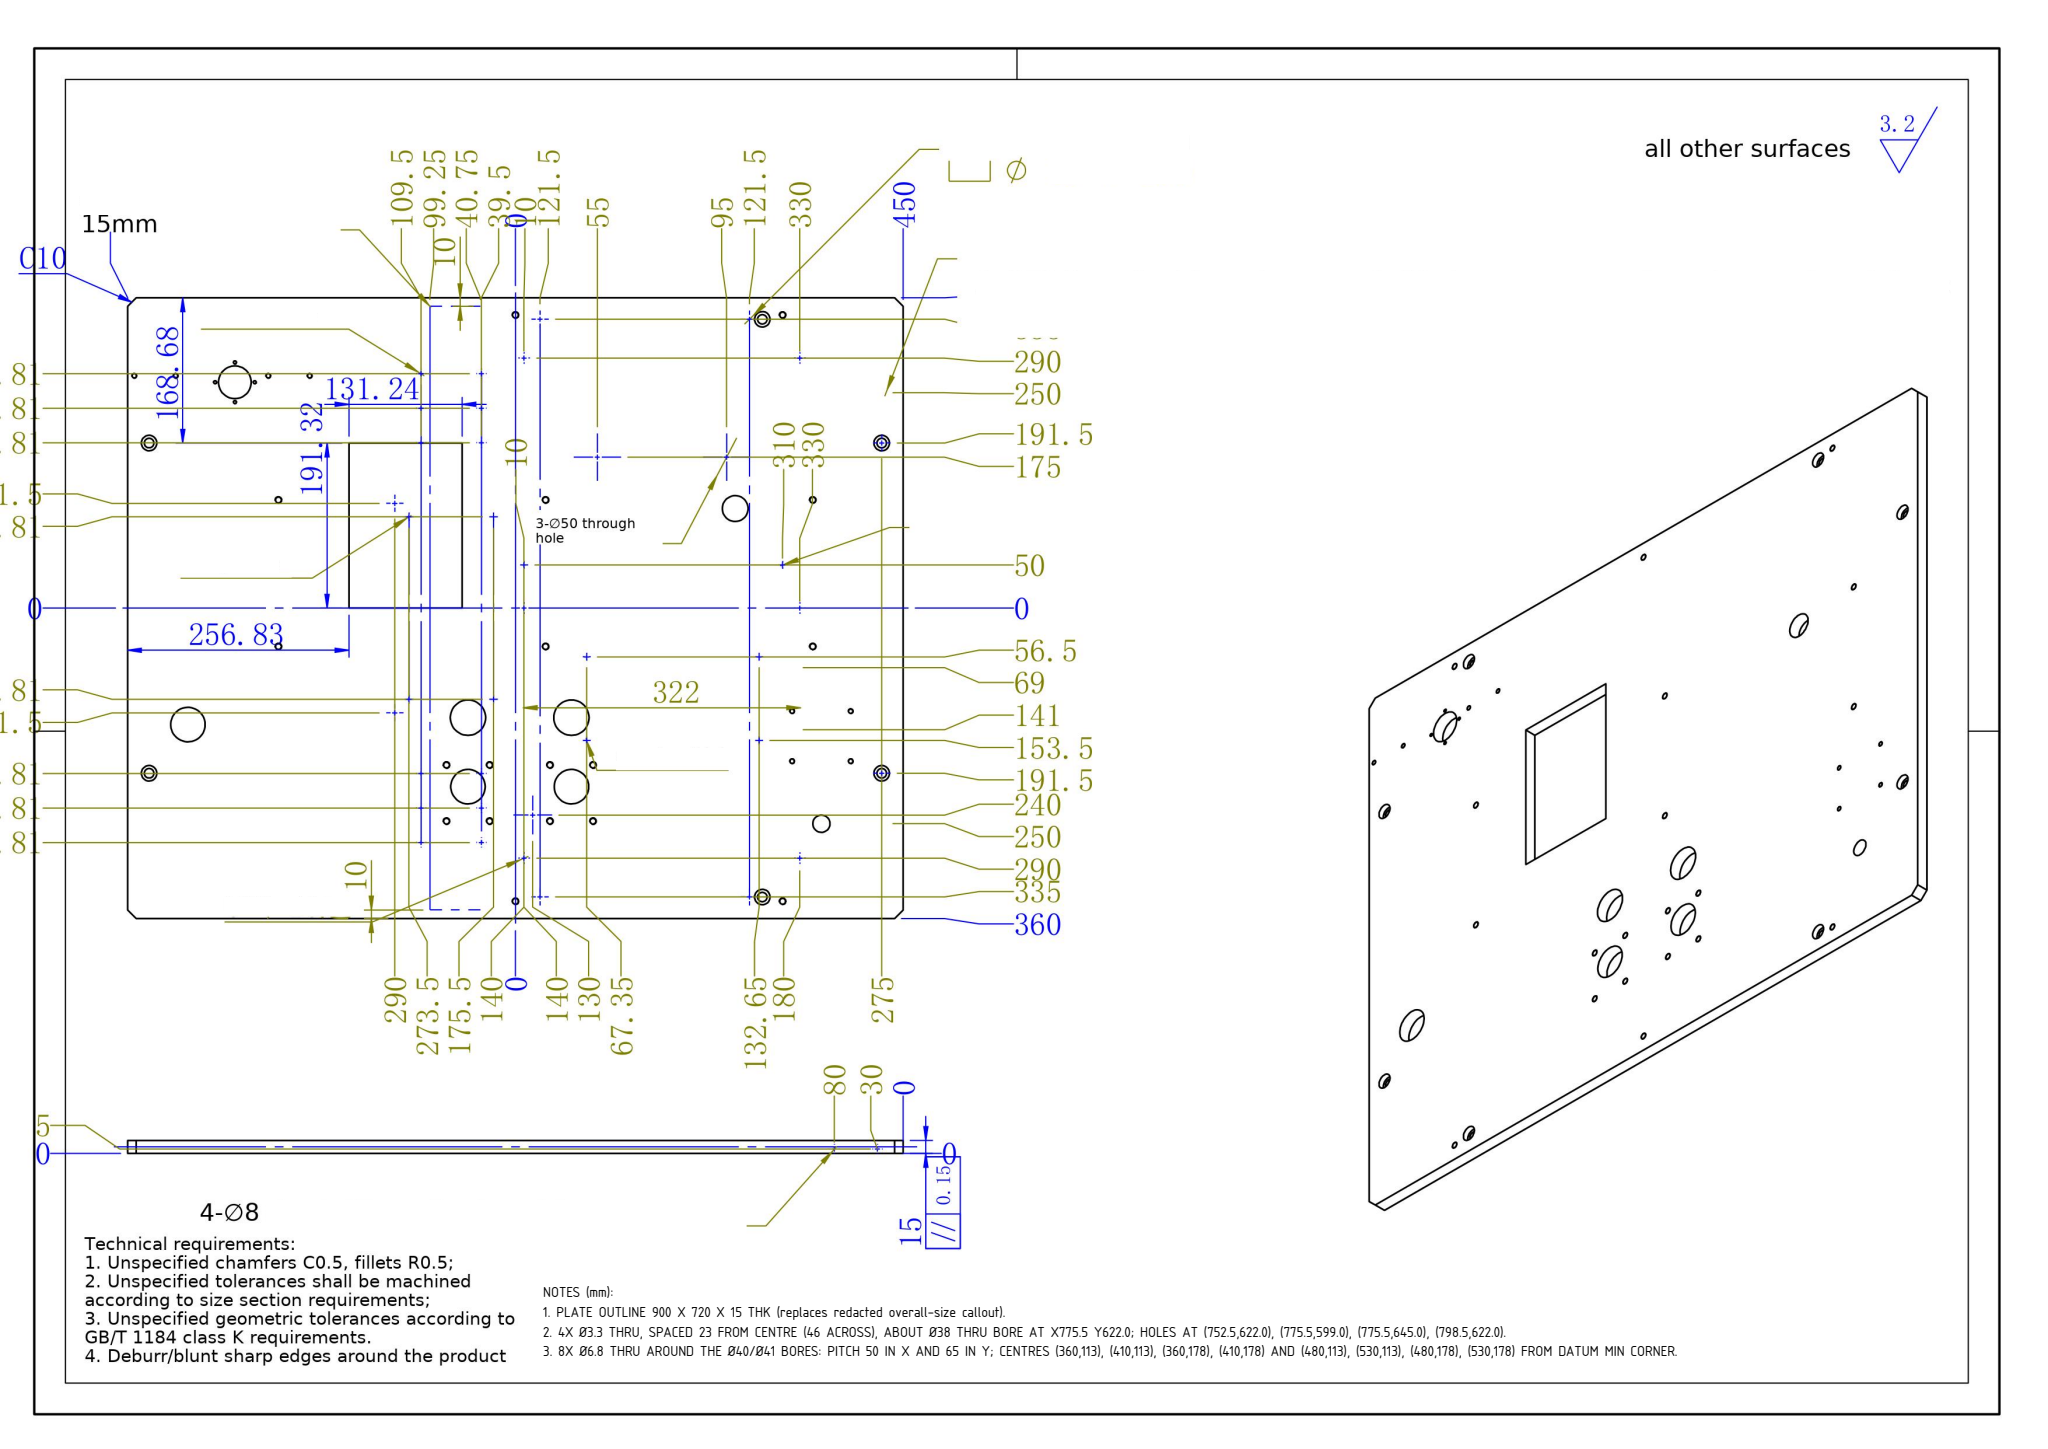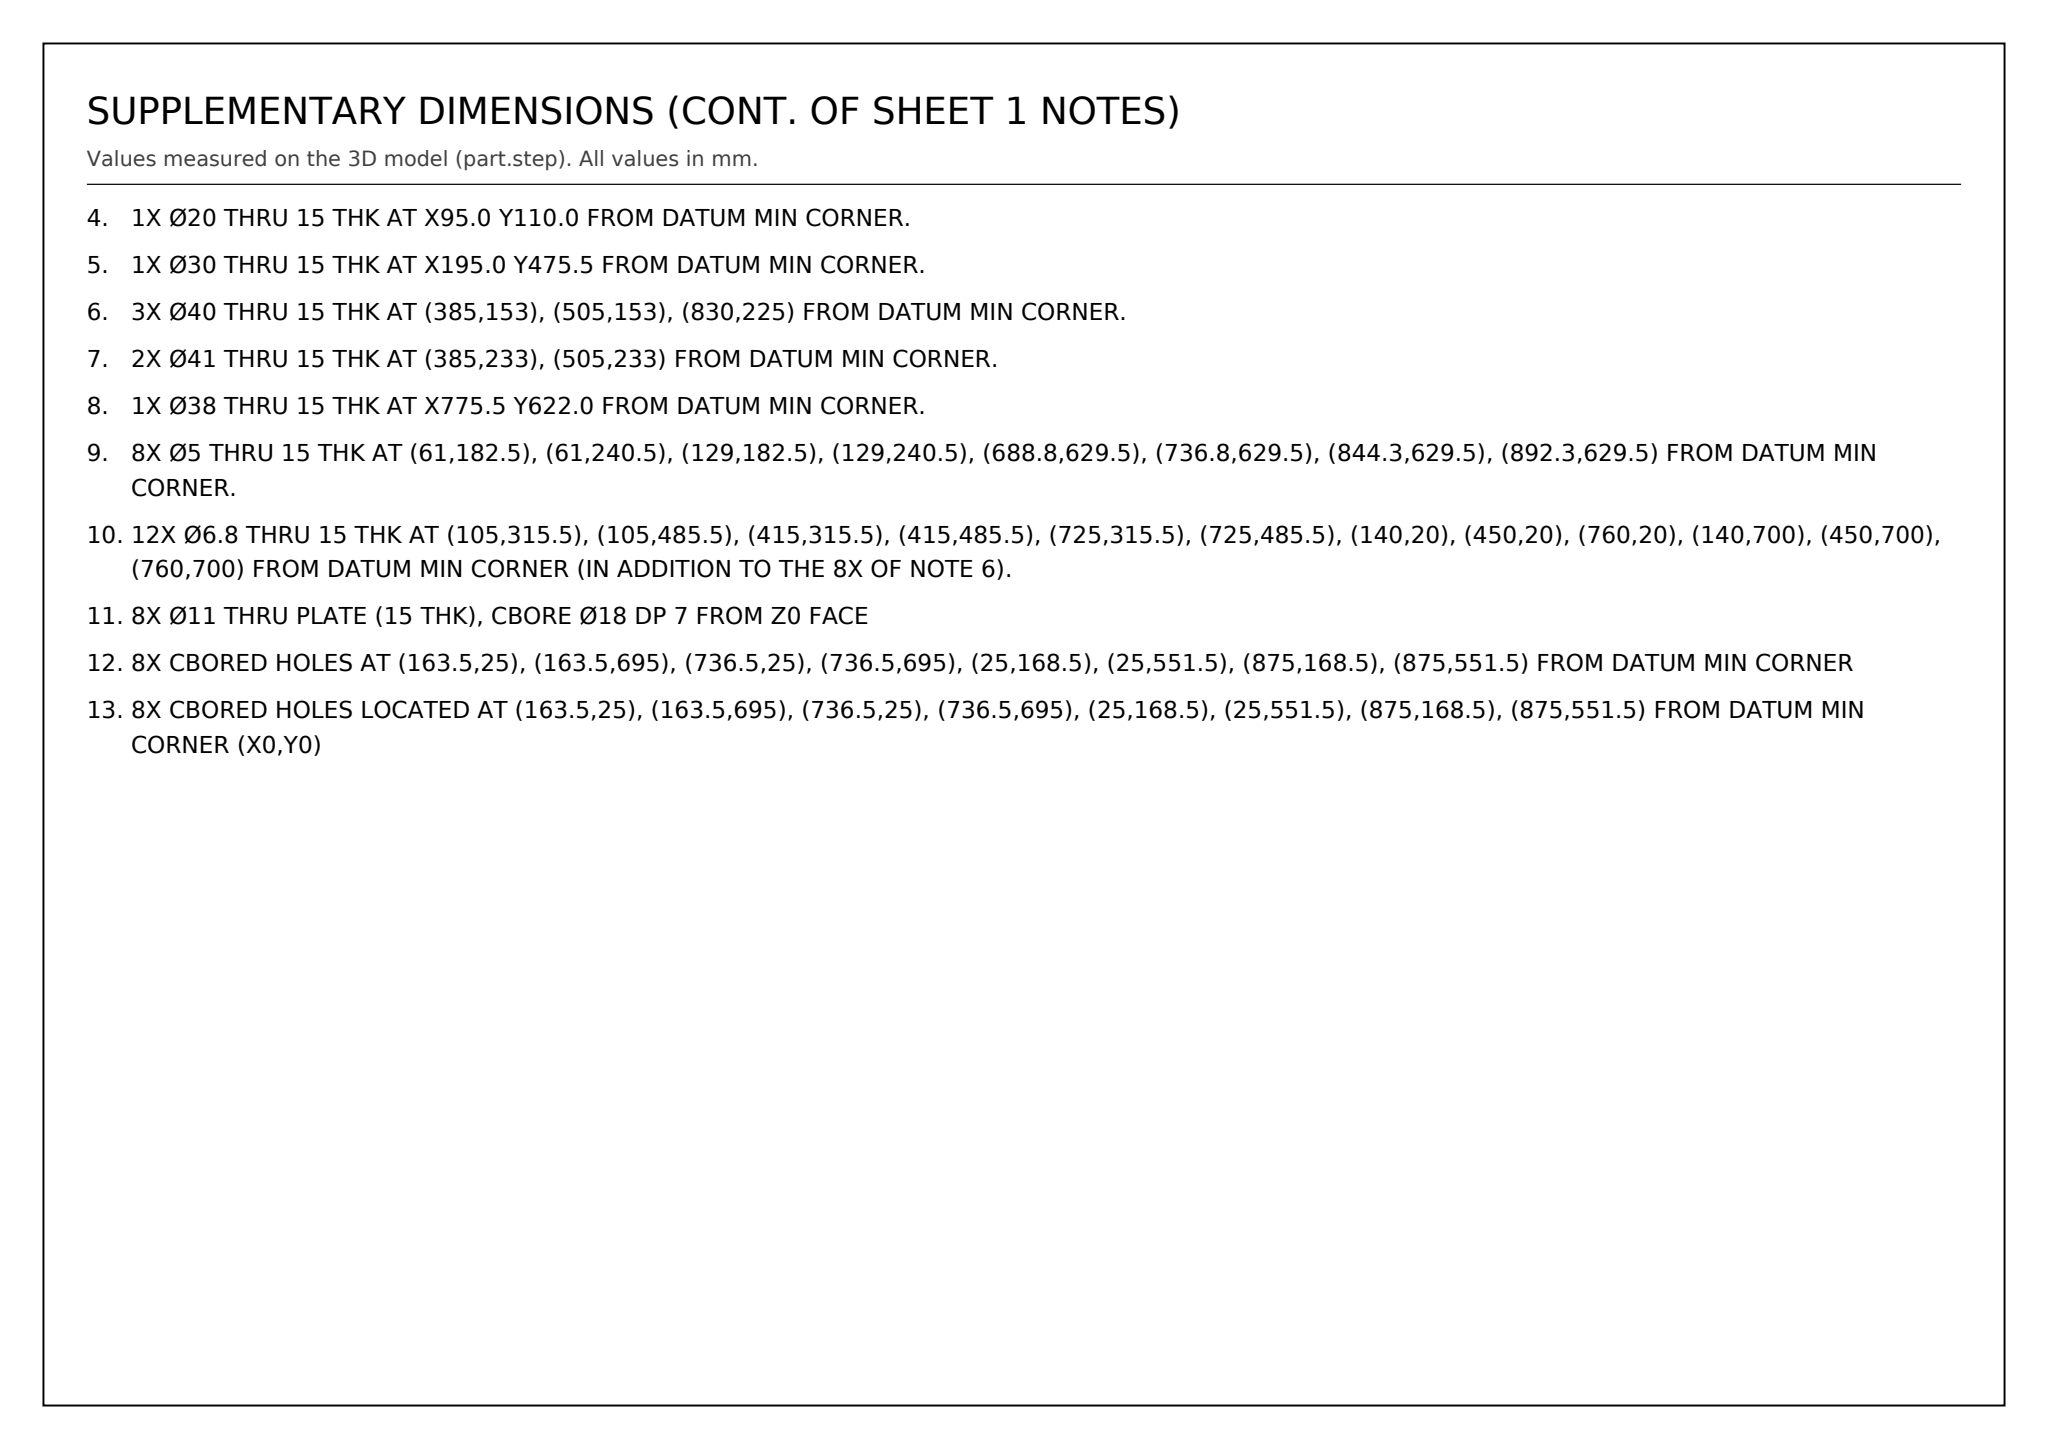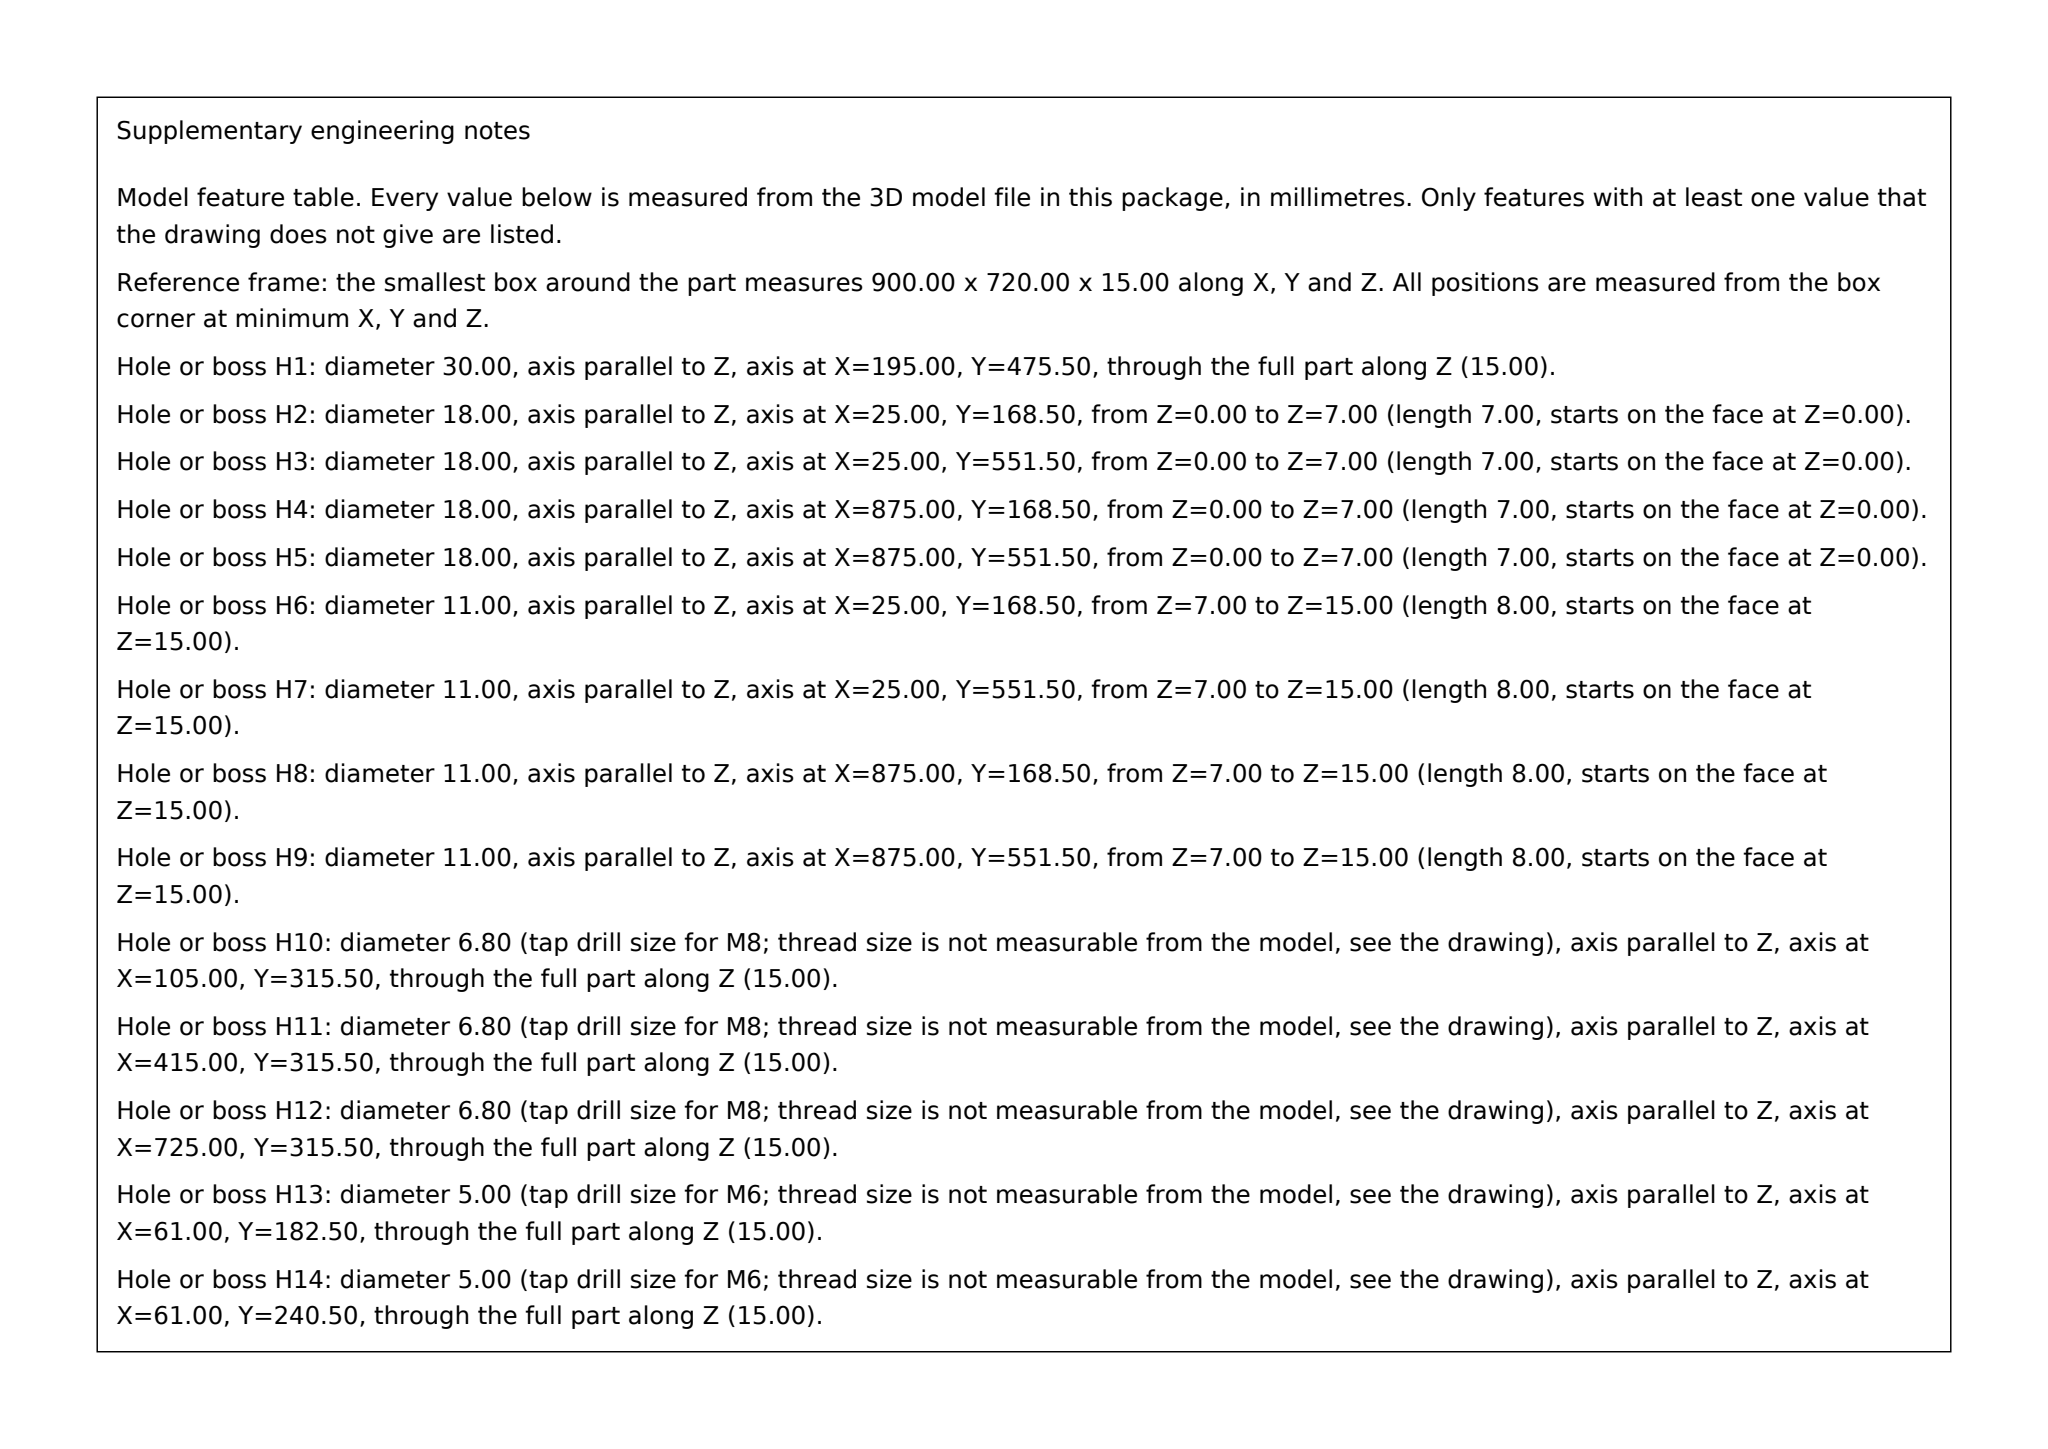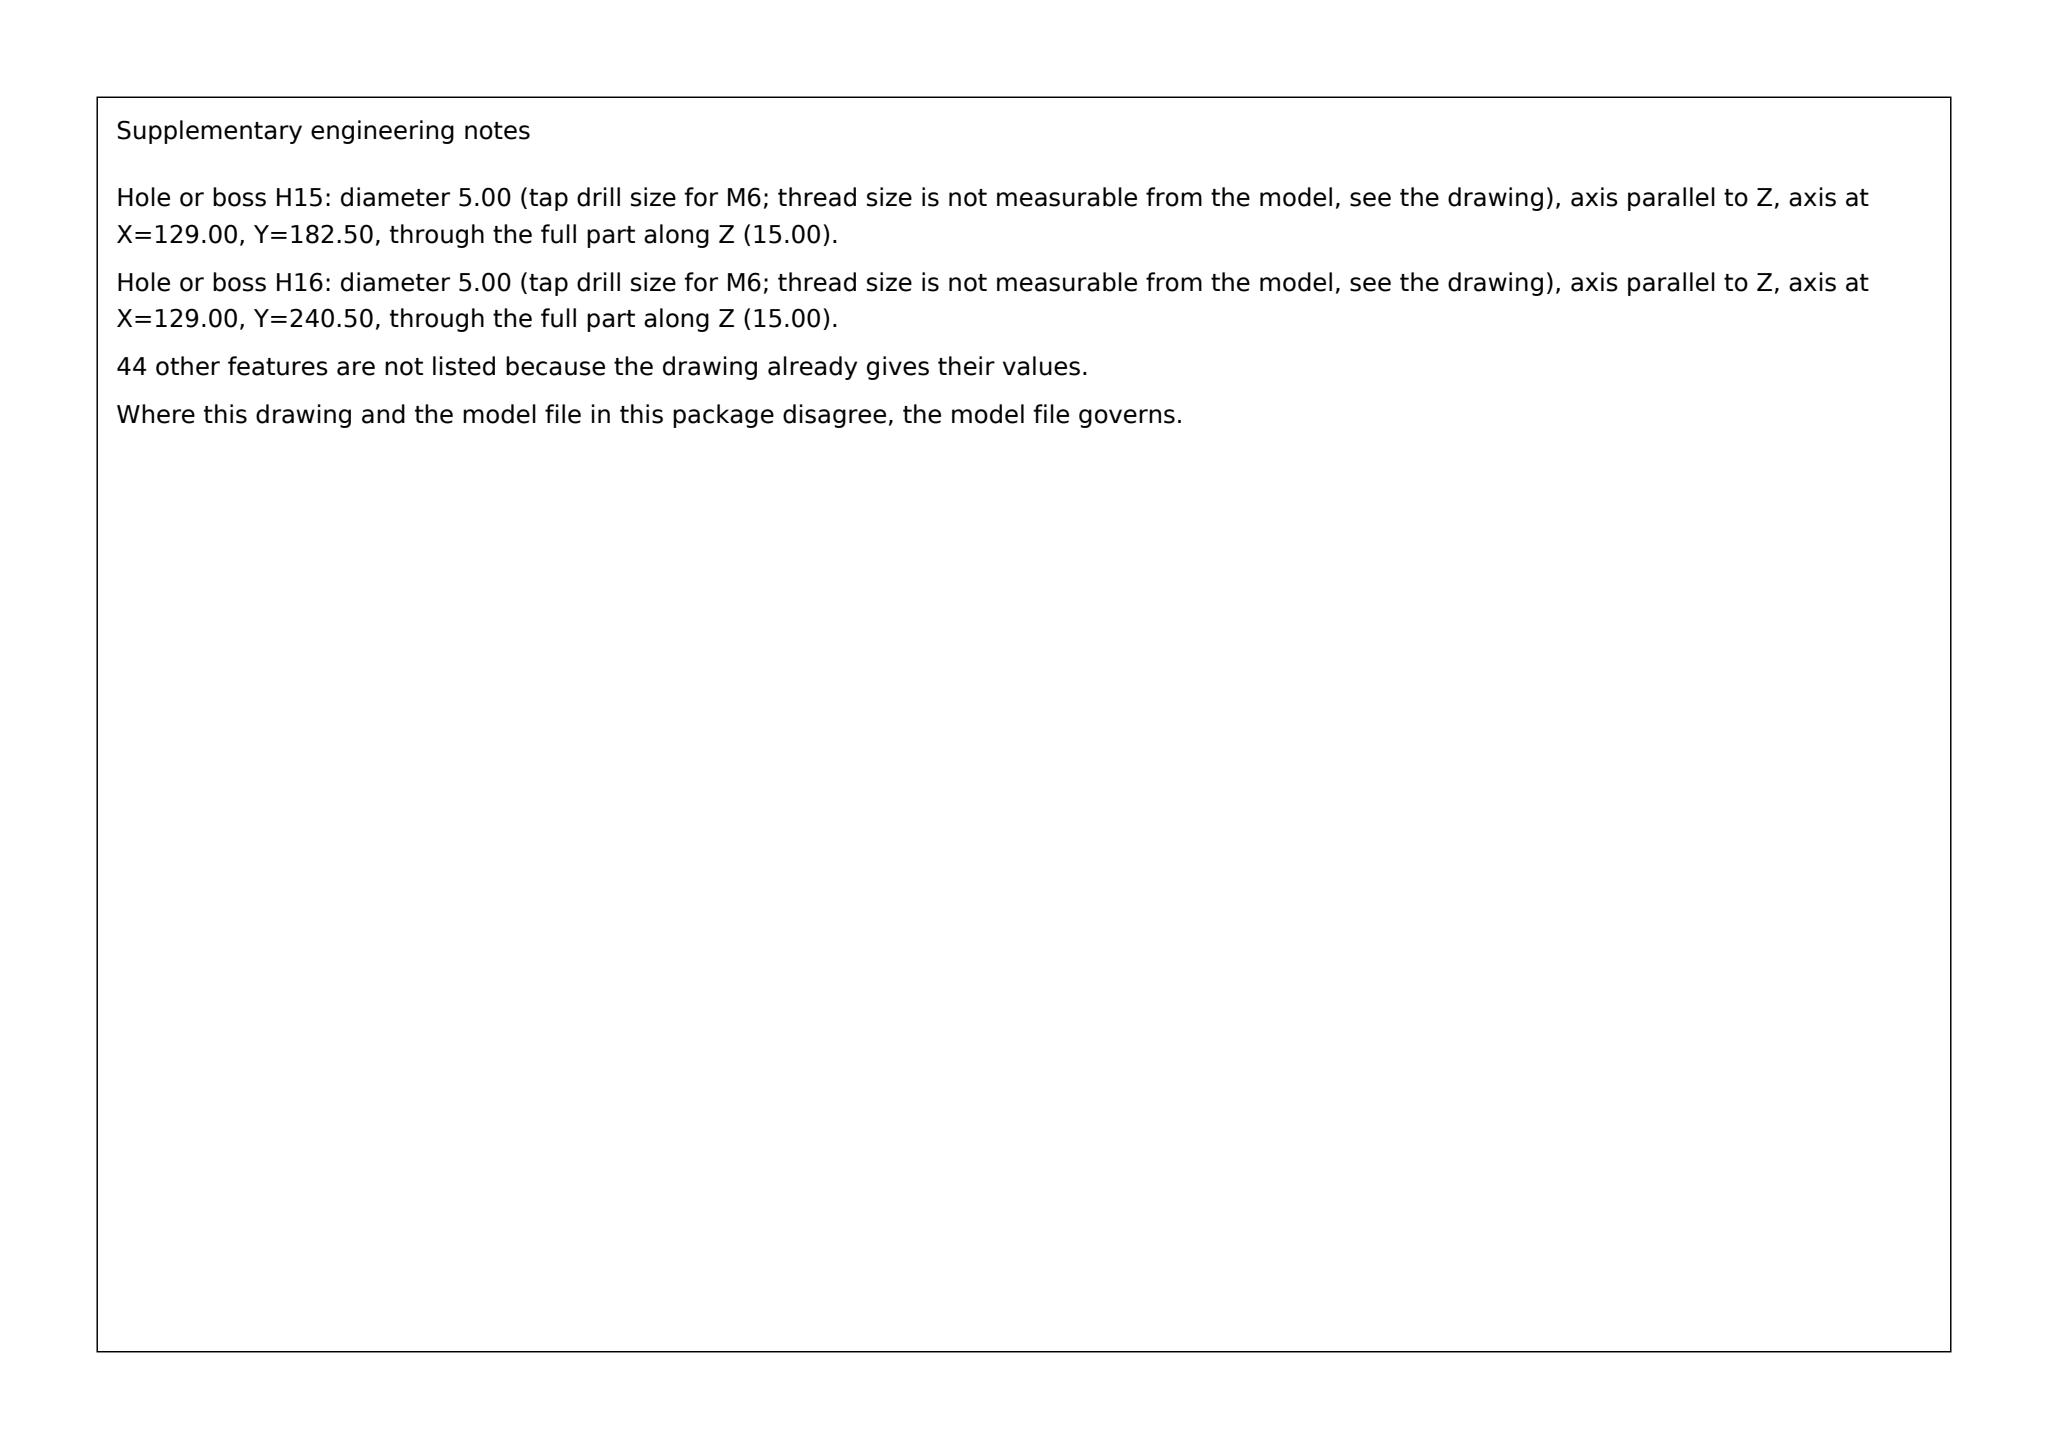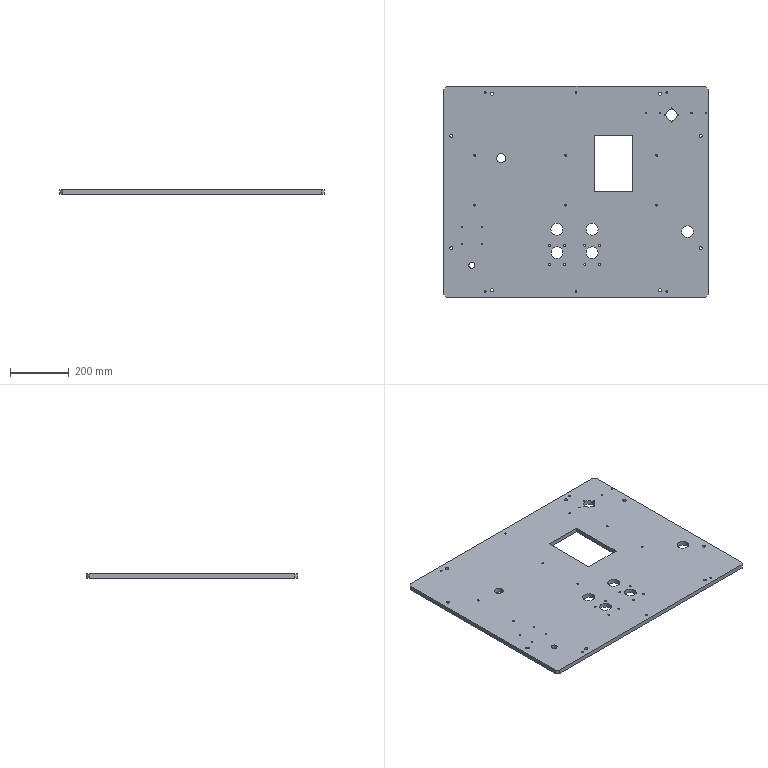Part | SolidWorks | mm | 1 solid | 134 faces | box 900 x 720 x 15 mm | volume 9177789 mm3 | cylinder 112 | plane 22 | commonest cylinder face diameters 6.8 x40 18 x16 11 x16 5 x16 3.3 x8 40 x6 41 x4 20 x2
Drawing notes:
PLATE OUTLINE 900 X 720 X 15 THK (replaces redacted overall-size callout). | from the solid: bbox_xyz = [900.0, 720.0, 15.0]
4X Ø3.3 THRU, SPACED 23 FROM CENTRE (46 ACROSS), ABOUT Ø38 THRU BORE AT X775.5 Y622.0; HOLES AT (752.5,622.0), (775.5,599.0), (775.5,645.0), (798.5,622.0). | from the solid: cylinders dia 3.3 z 0-15 at those four positions; cylinder dia 38.0 z 0-15 at (775.5,622.0)
8X Ø6.8 THRU AROUND THE Ø40/Ø41 BORES: PITCH 50 IN X AND 65 IN Y; CENTRES (360,113), (410,113), (360,178), (410,178) AND (480,113), (530,113), (480,178), (530,178) FROM DATUM MIN CORNER. | from the solid: cylinders dia 6.8 z 0-15 at (360/410/480/530, 113/178); cylinders dia 40.0/41.0 at (385,153), (505,153), (385,233), (505,233)
1X Ø20 THRU 15 THK AT X95.0 Y110.0 FROM DATUM MIN CORNER. | from the solid: cylinder dia 20.0 axis z at [95.0,110.0], from 0.0 to 15.0
1X Ø30 THRU 15 THK AT X195.0 Y475.5 FROM DATUM MIN CORNER. | from the solid: cylinder dia 30.0 axis z at [195.0,475.5], from 0.0 to 15.0
3X Ø40 THRU 15 THK AT (385,153), (505,153), (830,225) FROM DATUM MIN CORNER. | from the solid: cylinders dia 40.0 axis z at [385,153], [505,153], [830,225], from 0.0 to 15.0
2X Ø41 THRU 15 THK AT (385,233), (505,233) FROM DATUM MIN CORNER. | from the solid: cylinders dia 41.0 axis z at [385,233], [505,233], from 0.0 to 15.0
1X Ø38 THRU 15 THK AT X775.5 Y622.0 FROM DATUM MIN CORNER. | from the solid: cylinder dia 38.0 axis z at [775.5,622.0], from 0.0 to 15.0
8X Ø5 THRU 15 THK AT (61,182.5), (61,240.5), (129,182.5), (129,240.5), (688.8,629.5), (736.8,629.5), (844.3,629.5), (892.3,629.5) FROM DATUM MIN CORNER. | from the solid: cylinders dia 5.0 axis z at those eight x,y, from 0.0 to 15.0
12X Ø6.8 THRU 15 THK AT (105,315.5), (105,485.5), (415,315.5), (415,485.5), (725,315.5), (725,485.5), (140,20), (450,20), (760,20), (140,700), (450,700), (760,700) FROM DATUM MIN CORNER (IN ADDITION TO THE 8X OF NOTE 6). | from the solid: cylinders dia 6.8 axis z at those twelve x,y, from 0.0 to 15.0
8X Ø11 THRU PLATE (15 THK), CBORE Ø18 DP 7 FROM Z0 FACE | from the solid: cylinders dia 11.0 axis z from 7.0 to 15.0 (8 off) and dia 18.0 axis z from 0.0 to 7.0 (8 off); z=7.0 cbore bottom planes, 18x18 extents
8X CBORED HOLES AT (163.5,25), (163.5,695), (736.5,25), (736.5,695), (25,168.5), (25,551.5), (875,168.5), (875,551.5) FROM DATUM MIN CORNER | from the solid: cylinder axis positions of the dia 11.0 / dia 18.0 pairs (axis_pos x,y values)
8X CBORED HOLES LOCATED AT (163.5,25), (163.5,695), (736.5,25), (736.5,695), (25,168.5), (25,551.5), (875,168.5), (875,551.5) FROM DATUM MIN CORNER (X0,Y0) | from the solid: cylinder axis positions of the Ø11/Ø18 coaxial pairs: [163.5,25], [163.5,695], [736.5,25], [736.5,695], [25,168.5], [25,551.5], [875,168.5], [875,551.5]
build123d program:
from build123d import *

# Parameters (mm, degrees)
BOSS_EXTRUDE1_DEPTH                               = 15
CHAMFER1_SIZE                                     = 10
M8_TAPPED_HOLE1_D                                 = 6.8
M6_TAPPED_HOLE1_D                                 = 5
M4_TAPPED_HOLE1_D                                 = 3.3
SKETCH13_R                                        = 19
CUT_EXTRUDE1_DEPTH                                = 970.446
M6_TAPPED_HOLE2_D                                 = 5
M8_TAPPED_HOLE2_D                                 = 6.8
SKETCH18_R                                        = 20
CUT_EXTRUDE2_DEPTH                                = 970.446
HOLE_SIZE_ACCORDING_TO_HEXAGON_SOCKET_D           = 11
HOLE_SIZE_ACCORDING_TO_HEXAGON_SOCKET_CBORE_D     = 18
HOLE_SIZE_ACCORDING_TO_HEXAGON_SOCKET_CBORE_DEPTH = 7
SKETCH23_R                                        = 20.5
CUT_EXTRUDE3_DEPTH                                = 970.446
M8_TAPPED_HOLE3_D                                 = 6.8
SKETCH26_R                                        = 15
CUT_EXTRUDE4_DEPTH                                = 970.446
SKETCH27_R                                        = 10
CUT_EXTRUDE5_DEPTH                                = 970.446
SKETCH28_R                                        = 20
CUT_EXTRUDE6_DEPTH                                = 970.446
SKETCH29_W                                        = 131.236
SKETCH29_H                                        = 191.325
CUT_EXTRUDE7_DEPTH                                = 215


with BuildPart() as part:
    # Sketch1 → Boss-Extrude1 (new body)
    with BuildSketch(Plane.XY):
        Polygon((0, 0), (0, 360), (900, 360), (900, -360), (0, -360), align=None)
    extrude(amount=BOSS_EXTRUDE1_DEPTH)

    # Chamfer1
    chamfer1_edges = [part.edges().sort_by_distance(p)[0] for p in [
        (0, 360, 7.5),
        (900, 360, 7.5),
        (900, -360, 7.5),
        (0, -360, 7.5),
    ]]
    chamfer(chamfer1_edges, length=CHAMFER1_SIZE)

    # M8 Tapped Hole1 (through all)
    with Locations(Plane(origin=(0, 0, 0), x_dir=(-1, 0, 0), z_dir=(0, 0, -1))):
        with Locations((-725, 125.5), (-725, -44.5), (-415, -44.5), (-415, 125.5), (-105, 125.5), (-105, -44.5)):
            Hole(M8_TAPPED_HOLE1_D / 2)

    # M6 Tapped Hole1 (through all)
    with Locations(Plane(origin=(0, 0, 0), x_dir=(-1, 0, 0), z_dir=(0, 0, -1))):
        with Locations((-688.75, 269.45), (-736.75, 269.45), (-844.25, 269.45), (-892.25, 269.45)):
            Hole(M6_TAPPED_HOLE1_D / 2)

    # M4 Tapped Hole1 (through all)
    with Locations(Plane(origin=(0, 0, 0), x_dir=(-1, 0, 0), z_dir=(0, 0, -1))):
        with Locations((-798.5, 261.95), (-775.5, 284.95), (-752.5, 261.95), (-775.5, 238.95)):
            Hole(M4_TAPPED_HOLE1_D / 2)

    # Sketch13 → Cut-Extrude1 (cut, through all)
    with BuildSketch(Plane(origin=(0, 0, 0), x_dir=(-1, 0, 0), z_dir=(0, 0, -1))):
        with Locations((-775.5, 261.95)):
            Circle(SKETCH13_R)
    extrude(amount=-CUT_EXTRUDE1_DEPTH, mode=Mode.SUBTRACT)

    # M6 Tapped Hole2 (through all)
    with Locations(Plane(origin=(0, 0, 0), x_dir=(-1, 0, 0), z_dir=(0, 0, -1))):
        with Locations((-61, -177.5), (-61, -119.5), (-129, -177.5), (-129, -119.5)):
            Hole(M6_TAPPED_HOLE2_D / 2)

    # M8 Tapped Hole2 (through all)
    with Locations(Plane(origin=(0, 0, 0), x_dir=(-1, 0, 0), z_dir=(0, 0, -1))):
        with Locations((-480, -182), (-530, -182), (-480, -247), (-530, -247), (-410, -247), (-360, -247), (-410, -182), (-360, -182)):
            Hole(M8_TAPPED_HOLE2_D / 2)

    # Sketch18 → Cut-Extrude2 (cut, through all)
    with BuildSketch(Plane(origin=(0, 0, 0), x_dir=(-1, 0, 0), z_dir=(0, 0, -1))):
        with Locations((-505, -207)):
            Circle(SKETCH18_R)
        with Locations((-385, -207)):
            Circle(SKETCH18_R)
    extrude(amount=-CUT_EXTRUDE2_DEPTH, mode=Mode.SUBTRACT)

    # Hole Size _According to_ Hexagon Socket (through all)
    with Locations(Plane(origin=(0, 0, 0), x_dir=(-1, 0, 0), z_dir=(0, 0, -1))):
        with Locations((-736.5, 335), (-875, 191.5), (-875, -191.5), (-736.5, -335), (-163.5, -335), (-25, -191.5), (-25, 191.5), (-163.5, 335)):
            CounterBoreHole(HOLE_SIZE_ACCORDING_TO_HEXAGON_SOCKET_D / 2, HOLE_SIZE_ACCORDING_TO_HEXAGON_SOCKET_CBORE_D / 2, HOLE_SIZE_ACCORDING_TO_HEXAGON_SOCKET_CBORE_DEPTH)

    # Sketch23 → Cut-Extrude3 (cut, through all)
    with BuildSketch(Plane.XY.offset(15)):
        with Locations((385, -127)):
            Circle(SKETCH23_R)
        with Locations((505, -127)):
            Circle(SKETCH23_R)
    extrude(amount=-CUT_EXTRUDE3_DEPTH, mode=Mode.SUBTRACT)

    # M8 Tapped Hole3 (through all)
    with Locations(Plane(origin=(0, 0, 0), x_dir=(-1, 0, 0), z_dir=(0, 0, -1))):
        with Locations((-760, -340), (-140, -340), (-450, -340), (-760, 340), (-450, 340), (-140, 340)):
            Hole(M8_TAPPED_HOLE3_D / 2)

    # Sketch26 → Cut-Extrude4 (cut, through all)
    with BuildSketch(Plane(origin=(0, 0, 0), x_dir=(-1, 0, 0), z_dir=(0, 0, -1))):
        with Locations((-195, 115.5)):
            Circle(SKETCH26_R)
    extrude(amount=-CUT_EXTRUDE4_DEPTH, mode=Mode.SUBTRACT)

    # Sketch27 → Cut-Extrude5 (cut, through all)
    with BuildSketch(Plane(origin=(0, 0, 0), x_dir=(-1, 0, 0), z_dir=(0, 0, -1))):
        with Locations((-95, -250)):
            Circle(SKETCH27_R)
    extrude(amount=-CUT_EXTRUDE5_DEPTH, mode=Mode.SUBTRACT)

    # Sketch28 → Cut-Extrude6 (cut, through all)
    with BuildSketch(Plane(origin=(0, 0, 0), x_dir=(-1, 0, 0), z_dir=(0, 0, -1))):
        with Locations((-830, -135)):
            Circle(SKETCH28_R)
    extrude(amount=-CUT_EXTRUDE6_DEPTH, mode=Mode.SUBTRACT)

    # Sketch29 → Cut-Extrude7 (cut)
    with BuildSketch(Plane(origin=(0, 0, 0), x_dir=(-1, 0, 0), z_dir=(0, 0, -1))):
        with Locations((-577.55, 95.662)):
            Rectangle(SKETCH29_W, SKETCH29_H)
    extrude(amount=-CUT_EXTRUDE7_DEPTH, mode=Mode.SUBTRACT)


solid = part.part